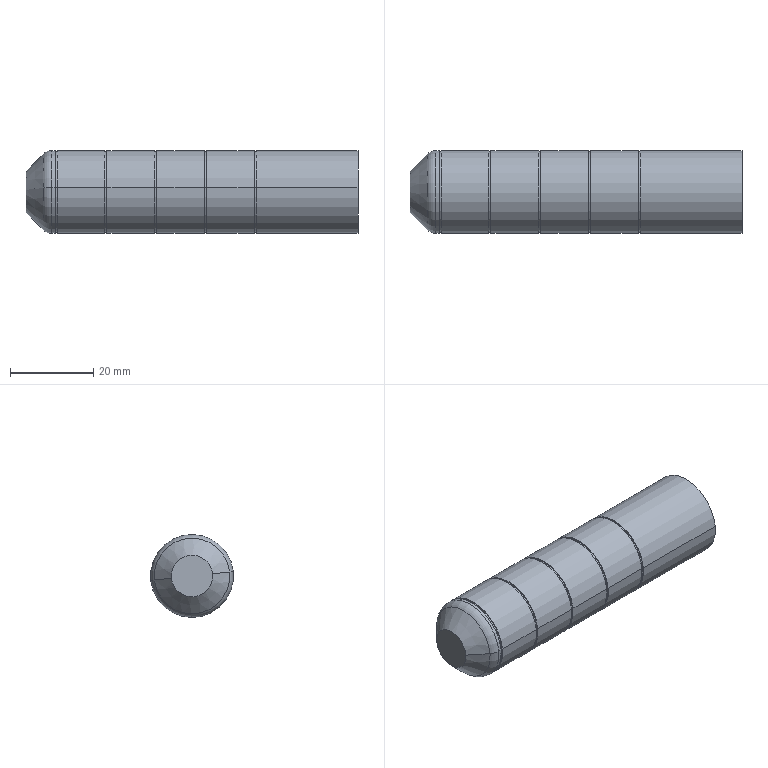Component | SolidWorks | ZN-A-018-2 | 1 solid | 42 faces | box 80 x 20 x 20 mm | volume 23686 mm3 | cylinder 24 | plane 12 | cone 4 | torus 2 | commonest cylinder face diameters 20 x12 19.5 x10 6.8 x2
STEP:
#1=COLOUR_RGB('',0.7922,0.8196,0.9333);
#2=FILL_AREA_STYLE_COLOUR('',#1);
#3=FILL_AREA_STYLE('',(#2));
#4=SURFACE_STYLE_FILL_AREA(#3);
#5=SURFACE_SIDE_STYLE('',(#4));
#6=SURFACE_STYLE_USAGE(.BOTH.,#5);
#7=PRESENTATION_STYLE_ASSIGNMENT((#6));
#8=CARTESIAN_POINT('',(14.356,6.199,4.014));
#9=VERTEX_POINT('',#8);
#10=CARTESIAN_POINT('',(14.356,5.416,4.097));
#11=VERTEX_POINT('',#10);
#12=CARTESIAN_POINT('',(14.356,5.807,4.055));
#13=DIRECTION('',(1.,-0.,0.));
#14=DIRECTION('',(0.,-0.9945,0.1051));
#15=AXIS2_PLACEMENT_3D('',#12,#13,#14);
#16=CIRCLE('',#15,0.3937);
#17=EDGE_CURVE('',#9,#11,#16,.T.);
#18=ORIENTED_EDGE('',*,*,#17,.T.);
#19=CARTESIAN_POINT('',(14.386,5.416,4.097));
#20=VERTEX_POINT('',#19);
#21=CARTESIAN_POINT('',(14.11,5.416,4.097));
#22=DIRECTION('',(1.,-0.,0.));
#23=VECTOR('',#22,39.37);
#24=LINE('',#21,#23);
#25=EDGE_CURVE('',#11,#20,#24,.T.);
#26=ORIENTED_EDGE('',*,*,#25,.T.);
#27=CARTESIAN_POINT('',(14.386,6.199,4.014));
#28=VERTEX_POINT('',#27);
#29=CARTESIAN_POINT('',(14.386,5.807,4.055));
#30=DIRECTION('',(1.,-0.,0.));
#31=DIRECTION('',(0.,0.9945,-0.1051));
#32=AXIS2_PLACEMENT_3D('',#29,#30,#31);
#33=CIRCLE('',#32,0.3937);
#34=EDGE_CURVE('',#28,#20,#33,.T.);
#35=ORIENTED_EDGE('',*,*,#34,.F.);
#36=CARTESIAN_POINT('',(14.11,6.199,4.014));
#37=DIRECTION('',(1.,-0.,0.));
#38=VECTOR('',#37,39.37);
#39=LINE('',#36,#38);
#40=EDGE_CURVE('',#9,#28,#39,.T.);
#41=ORIENTED_EDGE('',*,*,#40,.F.);
#42=EDGE_LOOP('',(#18,#26,#35,#41));
#43=FACE_OUTER_BOUND('',#42,.T.);
#44=CARTESIAN_POINT('',(14.11,5.807,4.055));
#45=DIRECTION('',(1.,-0.,0.));
#46=DIRECTION('',(0.,0.9945,-0.1051));
#47=AXIS2_PLACEMENT_3D('',#44,#45,#46);
#48=CYLINDRICAL_SURFACE('',#47,0.3937);
#49=ADVANCED_FACE('',(#43),#48,.T.);
#50=ORIENTED_EDGE('',*,*,#17,.F.);
#51=CARTESIAN_POINT('',(14.272,6.164,4.017));
#52=VERTEX_POINT('',#51);
#53=CARTESIAN_POINT('',(14.356,6.081,4.026));
#54=DIRECTION('',(-0.,0.1051,0.9945));
#55=DIRECTION('',(0.,-0.9945,0.1051));
#56=AXIS2_PLACEMENT_3D('',#53,#54,#55);
#57=CIRCLE('',#56,0.1181);
#58=EDGE_CURVE('',#9,#52,#57,.T.);
#59=ORIENTED_EDGE('',*,*,#58,.T.);
#60=CARTESIAN_POINT('',(14.272,5.45,4.093));
#61=VERTEX_POINT('',#60);
#62=CARTESIAN_POINT('',(14.272,5.807,4.055));
#63=DIRECTION('',(-1.,0.,-0.));
#64=DIRECTION('',(0.,0.9945,-0.1051));
#65=AXIS2_PLACEMENT_3D('',#62,#63,#64);
#66=CIRCLE('',#65,0.3591);
#67=EDGE_CURVE('',#61,#52,#66,.T.);
#68=ORIENTED_EDGE('',*,*,#67,.F.);
#69=CARTESIAN_POINT('',(14.356,5.533,4.084));
#70=DIRECTION('',(0.,-0.1051,-0.9945));
#71=DIRECTION('',(0.,0.9945,-0.1051));
#72=AXIS2_PLACEMENT_3D('',#69,#70,#71);
#73=CIRCLE('',#72,0.1181);
#74=EDGE_CURVE('',#11,#61,#73,.T.);
#75=ORIENTED_EDGE('',*,*,#74,.F.);
#76=EDGE_LOOP('',(#50,#59,#68,#75));
#77=FACE_OUTER_BOUND('',#76,.T.);
#78=CARTESIAN_POINT('',(14.356,5.807,4.055));
#79=DIRECTION('',(-1.,0.,-0.));
#80=DIRECTION('',(-0.,-0.9945,0.1051));
#81=AXIS2_PLACEMENT_3D('',#78,#79,#80);
#82=TOROIDAL_SURFACE('',#81,0.2756,0.1181);
#83=ADVANCED_FACE('',(#77),#82,.T.);
#84=CARTESIAN_POINT('',(14.11,5.611,4.076));
#85=VERTEX_POINT('',#84);
#86=CARTESIAN_POINT('',(14.11,6.003,4.034));
#87=VERTEX_POINT('',#86);
#88=CARTESIAN_POINT('',(14.11,5.807,4.055));
#89=DIRECTION('',(-1.,0.,-0.));
#90=DIRECTION('',(0.,-0.9945,0.1051));
#91=AXIS2_PLACEMENT_3D('',#88,#89,#90);
#92=CIRCLE('',#91,0.1969);
#93=EDGE_CURVE('',#85,#87,#92,.T.);
#94=ORIENTED_EDGE('',*,*,#93,.F.);
#95=CARTESIAN_POINT('',(14.11,5.611,4.076));
#96=DIRECTION('',(0.7071,-0.7032,0.07433));
#97=VECTOR('',#96,39.37);
#98=LINE('',#95,#97);
#99=EDGE_CURVE('',#85,#61,#98,.T.);
#100=ORIENTED_EDGE('',*,*,#99,.T.);
#101=ORIENTED_EDGE('',*,*,#67,.T.);
#102=CARTESIAN_POINT('',(14.11,6.003,4.034));
#103=DIRECTION('',(0.7071,0.7032,-0.07433));
#104=VECTOR('',#103,39.37);
#105=LINE('',#102,#104);
#106=EDGE_CURVE('',#87,#52,#105,.T.);
#107=ORIENTED_EDGE('',*,*,#106,.F.);
#108=EDGE_LOOP('',(#94,#100,#101,#107));
#109=FACE_OUTER_BOUND('',#108,.T.);
#110=CARTESIAN_POINT('',(14.11,5.807,4.055));
#111=DIRECTION('',(1.,-0.,0.));
#112=DIRECTION('',(0.,0.9945,-0.1051));
#113=AXIS2_PLACEMENT_3D('',#110,#111,#112);
#114=CONICAL_SURFACE('',#113,0.1969,0.7854);
#115=ADVANCED_FACE('',(#109),#114,.T.);
#116=CARTESIAN_POINT('',(14.405,6.189,4.015));
#117=VERTEX_POINT('',#116);
#118=CARTESIAN_POINT('',(14.405,5.425,4.095));
#119=VERTEX_POINT('',#118);
#120=CARTESIAN_POINT('',(14.405,5.807,4.055));
#121=DIRECTION('',(1.,-0.,0.));
#122=DIRECTION('',(0.,0.9945,-0.1051));
#123=AXIS2_PLACEMENT_3D('',#120,#121,#122);
#124=CIRCLE('',#123,0.3839);
#125=EDGE_CURVE('',#117,#119,#124,.T.);
#126=ORIENTED_EDGE('',*,*,#125,.F.);
#127=CARTESIAN_POINT('',(14.386,6.189,4.015));
#128=VERTEX_POINT('',#127);
#129=CARTESIAN_POINT('',(14.405,6.189,4.015));
#130=DIRECTION('',(-1.,0.,-0.));
#131=VECTOR('',#130,39.37);
#132=LINE('',#129,#131);
#133=EDGE_CURVE('',#117,#128,#132,.T.);
#134=ORIENTED_EDGE('',*,*,#133,.T.);
#135=CARTESIAN_POINT('',(14.386,5.425,4.095));
#136=VERTEX_POINT('',#135);
#137=CARTESIAN_POINT('',(14.386,5.807,4.055));
#138=DIRECTION('',(1.,-0.,0.));
#139=DIRECTION('',(0.,0.9945,-0.1051));
#140=AXIS2_PLACEMENT_3D('',#137,#138,#139);
#141=CIRCLE('',#140,0.3839);
#142=EDGE_CURVE('',#128,#136,#141,.T.);
#143=ORIENTED_EDGE('',*,*,#142,.T.);
#144=CARTESIAN_POINT('',(14.405,5.425,4.095));
#145=DIRECTION('',(-1.,0.,-0.));
#146=VECTOR('',#145,39.37);
#147=LINE('',#144,#146);
#148=EDGE_CURVE('',#119,#136,#147,.T.);
#149=ORIENTED_EDGE('',*,*,#148,.F.);
#150=EDGE_LOOP('',(#126,#134,#143,#149));
#151=FACE_OUTER_BOUND('',#150,.T.);
#152=CARTESIAN_POINT('',(14.405,5.807,4.055));
#153=DIRECTION('',(-1.,0.,-0.));
#154=DIRECTION('',(0.,-0.9945,0.1051));
#155=AXIS2_PLACEMENT_3D('',#152,#153,#154);
#156=CYLINDRICAL_SURFACE('',#155,0.3839);
#157=ADVANCED_FACE('',(#151),#156,.T.);
#158=CARTESIAN_POINT('',(14.405,6.199,4.014));
#159=VERTEX_POINT('',#158);
#160=CARTESIAN_POINT('',(14.405,5.416,4.097));
#161=VERTEX_POINT('',#160);
#162=CARTESIAN_POINT('',(14.405,5.807,4.055));
#163=DIRECTION('',(1.,-0.,0.));
#164=DIRECTION('',(0.,0.9945,-0.1051));
#165=AXIS2_PLACEMENT_3D('',#162,#163,#164);
#166=CIRCLE('',#165,0.3937);
#167=EDGE_CURVE('',#159,#161,#166,.T.);
#168=ORIENTED_EDGE('',*,*,#167,.T.);
#169=CARTESIAN_POINT('',(14.858,5.416,4.097));
#170=VERTEX_POINT('',#169);
#171=CARTESIAN_POINT('',(14.11,5.416,4.097));
#172=DIRECTION('',(1.,-0.,0.));
#173=VECTOR('',#172,39.37);
#174=LINE('',#171,#173);
#175=EDGE_CURVE('',#161,#170,#174,.T.);
#176=ORIENTED_EDGE('',*,*,#175,.T.);
#177=CARTESIAN_POINT('',(14.858,6.199,4.014));
#178=VERTEX_POINT('',#177);
#179=CARTESIAN_POINT('',(14.858,5.807,4.055));
#180=DIRECTION('',(1.,-0.,0.));
#181=DIRECTION('',(0.,0.9945,-0.1051));
#182=AXIS2_PLACEMENT_3D('',#179,#180,#181);
#183=CIRCLE('',#182,0.3937);
#184=EDGE_CURVE('',#178,#170,#183,.T.);
#185=ORIENTED_EDGE('',*,*,#184,.F.);
#186=CARTESIAN_POINT('',(14.11,6.199,4.014));
#187=DIRECTION('',(1.,-0.,0.));
#188=VECTOR('',#187,39.37);
#189=LINE('',#186,#188);
#190=EDGE_CURVE('',#159,#178,#189,.T.);
#191=ORIENTED_EDGE('',*,*,#190,.F.);
#192=EDGE_LOOP('',(#168,#176,#185,#191));
#193=FACE_OUTER_BOUND('',#192,.T.);
#194=CARTESIAN_POINT('',(14.11,5.807,4.055));
#195=DIRECTION('',(1.,-0.,0.));
#196=DIRECTION('',(0.,0.9945,-0.1051));
#197=AXIS2_PLACEMENT_3D('',#194,#195,#196);
#198=CYLINDRICAL_SURFACE('',#197,0.3937);
#199=ADVANCED_FACE('',(#193),#198,.T.);
#200=CARTESIAN_POINT('',(14.878,6.189,4.015));
#201=VERTEX_POINT('',#200);
#202=CARTESIAN_POINT('',(14.878,5.425,4.095));
#203=VERTEX_POINT('',#202);
#204=CARTESIAN_POINT('',(14.878,5.807,4.055));
#205=DIRECTION('',(1.,-0.,0.));
#206=DIRECTION('',(0.,0.9945,-0.1051));
#207=AXIS2_PLACEMENT_3D('',#204,#205,#206);
#208=CIRCLE('',#207,0.3839);
#209=EDGE_CURVE('',#201,#203,#208,.T.);
#210=ORIENTED_EDGE('',*,*,#209,.F.);
#211=CARTESIAN_POINT('',(14.858,6.189,4.015));
#212=VERTEX_POINT('',#211);
#213=CARTESIAN_POINT('',(14.878,6.189,4.015));
#214=DIRECTION('',(-1.,0.,-0.));
#215=VECTOR('',#214,39.37);
#216=LINE('',#213,#215);
#217=EDGE_CURVE('',#201,#212,#216,.T.);
#218=ORIENTED_EDGE('',*,*,#217,.T.);
#219=CARTESIAN_POINT('',(14.858,5.425,4.095));
#220=VERTEX_POINT('',#219);
#221=CARTESIAN_POINT('',(14.858,5.807,4.055));
#222=DIRECTION('',(1.,-0.,0.));
#223=DIRECTION('',(0.,0.9945,-0.1051));
#224=AXIS2_PLACEMENT_3D('',#221,#222,#223);
#225=CIRCLE('',#224,0.3839);
#226=EDGE_CURVE('',#212,#220,#225,.T.);
#227=ORIENTED_EDGE('',*,*,#226,.T.);
#228=CARTESIAN_POINT('',(14.878,5.425,4.095));
#229=DIRECTION('',(-1.,0.,-0.));
#230=VECTOR('',#229,39.37);
#231=LINE('',#228,#230);
#232=EDGE_CURVE('',#203,#220,#231,.T.);
#233=ORIENTED_EDGE('',*,*,#232,.F.);
#234=EDGE_LOOP('',(#210,#218,#227,#233));
#235=FACE_OUTER_BOUND('',#234,.T.);
#236=CARTESIAN_POINT('',(14.878,5.807,4.055));
#237=DIRECTION('',(-1.,0.,-0.));
#238=DIRECTION('',(0.,-0.9945,0.1051));
#239=AXIS2_PLACEMENT_3D('',#236,#237,#238);
#240=CYLINDRICAL_SURFACE('',#239,0.3839);
#241=ADVANCED_FACE('',(#235),#240,.T.);
#242=CARTESIAN_POINT('',(14.878,6.199,4.014));
#243=VERTEX_POINT('',#242);
#244=CARTESIAN_POINT('',(14.878,5.416,4.097));
#245=VERTEX_POINT('',#244);
#246=CARTESIAN_POINT('',(14.878,5.807,4.055));
#247=DIRECTION('',(1.,-0.,0.));
#248=DIRECTION('',(0.,0.9945,-0.1051));
#249=AXIS2_PLACEMENT_3D('',#246,#247,#248);
#250=CIRCLE('',#249,0.3937);
#251=EDGE_CURVE('',#243,#245,#250,.T.);
#252=ORIENTED_EDGE('',*,*,#251,.T.);
#253=CARTESIAN_POINT('',(15.33,5.416,4.097));
#254=VERTEX_POINT('',#253);
#255=CARTESIAN_POINT('',(14.11,5.416,4.097));
#256=DIRECTION('',(1.,-0.,0.));
#257=VECTOR('',#256,39.37);
#258=LINE('',#255,#257);
#259=EDGE_CURVE('',#245,#254,#258,.T.);
#260=ORIENTED_EDGE('',*,*,#259,.T.);
#261=CARTESIAN_POINT('',(15.33,6.199,4.014));
#262=VERTEX_POINT('',#261);
#263=CARTESIAN_POINT('',(15.33,5.807,4.055));
#264=DIRECTION('',(1.,-0.,0.));
#265=DIRECTION('',(0.,0.9945,-0.1051));
#266=AXIS2_PLACEMENT_3D('',#263,#264,#265);
#267=CIRCLE('',#266,0.3937);
#268=EDGE_CURVE('',#262,#254,#267,.T.);
#269=ORIENTED_EDGE('',*,*,#268,.F.);
#270=CARTESIAN_POINT('',(14.11,6.199,4.014));
#271=DIRECTION('',(1.,-0.,0.));
#272=VECTOR('',#271,39.37);
#273=LINE('',#270,#272);
#274=EDGE_CURVE('',#243,#262,#273,.T.);
#275=ORIENTED_EDGE('',*,*,#274,.F.);
#276=EDGE_LOOP('',(#252,#260,#269,#275));
#277=FACE_OUTER_BOUND('',#276,.T.);
#278=CARTESIAN_POINT('',(14.11,5.807,4.055));
#279=DIRECTION('',(1.,-0.,0.));
#280=DIRECTION('',(0.,0.9945,-0.1051));
#281=AXIS2_PLACEMENT_3D('',#278,#279,#280);
#282=CYLINDRICAL_SURFACE('',#281,0.3937);
#283=ADVANCED_FACE('',(#277),#282,.T.);
#284=CARTESIAN_POINT('',(15.35,6.189,4.015));
#285=VERTEX_POINT('',#284);
#286=CARTESIAN_POINT('',(15.35,5.425,4.095));
#287=VERTEX_POINT('',#286);
#288=CARTESIAN_POINT('',(15.35,5.807,4.055));
#289=DIRECTION('',(1.,-0.,0.));
#290=DIRECTION('',(0.,0.9945,-0.1051));
#291=AXIS2_PLACEMENT_3D('',#288,#289,#290);
#292=CIRCLE('',#291,0.3839);
#293=EDGE_CURVE('',#285,#287,#292,.T.);
#294=ORIENTED_EDGE('',*,*,#293,.F.);
#295=CARTESIAN_POINT('',(15.33,6.189,4.015));
#296=VERTEX_POINT('',#295);
#297=CARTESIAN_POINT('',(15.35,6.189,4.015));
#298=DIRECTION('',(-1.,0.,-0.));
#299=VECTOR('',#298,39.37);
#300=LINE('',#297,#299);
#301=EDGE_CURVE('',#285,#296,#300,.T.);
#302=ORIENTED_EDGE('',*,*,#301,.T.);
#303=CARTESIAN_POINT('',(15.33,5.425,4.095));
#304=VERTEX_POINT('',#303);
#305=CARTESIAN_POINT('',(15.33,5.807,4.055));
#306=DIRECTION('',(1.,-0.,0.));
#307=DIRECTION('',(0.,0.9945,-0.1051));
#308=AXIS2_PLACEMENT_3D('',#305,#306,#307);
#309=CIRCLE('',#308,0.3839);
#310=EDGE_CURVE('',#296,#304,#309,.T.);
#311=ORIENTED_EDGE('',*,*,#310,.T.);
#312=CARTESIAN_POINT('',(15.35,5.425,4.095));
#313=DIRECTION('',(-1.,0.,-0.));
#314=VECTOR('',#313,39.37);
#315=LINE('',#312,#314);
#316=EDGE_CURVE('',#287,#304,#315,.T.);
#317=ORIENTED_EDGE('',*,*,#316,.F.);
#318=EDGE_LOOP('',(#294,#302,#311,#317));
#319=FACE_OUTER_BOUND('',#318,.T.);
#320=CARTESIAN_POINT('',(15.35,5.807,4.055));
#321=DIRECTION('',(-1.,0.,-0.));
#322=DIRECTION('',(0.,-0.9945,0.1051));
#323=AXIS2_PLACEMENT_3D('',#320,#321,#322);
#324=CYLINDRICAL_SURFACE('',#323,0.3839);
#325=ADVANCED_FACE('',(#319),#324,.T.);
#326=CARTESIAN_POINT('',(15.35,6.199,4.014));
#327=VERTEX_POINT('',#326);
#328=CARTESIAN_POINT('',(15.35,5.416,4.097));
#329=VERTEX_POINT('',#328);
#330=CARTESIAN_POINT('',(15.35,5.807,4.055));
#331=DIRECTION('',(1.,-0.,0.));
#332=DIRECTION('',(0.,0.9945,-0.1051));
#333=AXIS2_PLACEMENT_3D('',#330,#331,#332);
#334=CIRCLE('',#333,0.3937);
#335=EDGE_CURVE('',#327,#329,#334,.T.);
#336=ORIENTED_EDGE('',*,*,#335,.T.);
#337=CARTESIAN_POINT('',(15.803,5.416,4.097));
#338=VERTEX_POINT('',#337);
#339=CARTESIAN_POINT('',(14.11,5.416,4.097));
#340=DIRECTION('',(1.,-0.,0.));
#341=VECTOR('',#340,39.37);
#342=LINE('',#339,#341);
#343=EDGE_CURVE('',#329,#338,#342,.T.);
#344=ORIENTED_EDGE('',*,*,#343,.T.);
#345=CARTESIAN_POINT('',(15.803,6.199,4.014));
#346=VERTEX_POINT('',#345);
#347=CARTESIAN_POINT('',(15.803,5.807,4.055));
#348=DIRECTION('',(1.,-0.,0.));
#349=DIRECTION('',(0.,0.9945,-0.1051));
#350=AXIS2_PLACEMENT_3D('',#347,#348,#349);
#351=CIRCLE('',#350,0.3937);
#352=EDGE_CURVE('',#346,#338,#351,.T.);
#353=ORIENTED_EDGE('',*,*,#352,.F.);
#354=CARTESIAN_POINT('',(14.11,6.199,4.014));
#355=DIRECTION('',(1.,-0.,0.));
#356=VECTOR('',#355,39.37);
#357=LINE('',#354,#356);
#358=EDGE_CURVE('',#327,#346,#357,.T.);
#359=ORIENTED_EDGE('',*,*,#358,.F.);
#360=EDGE_LOOP('',(#336,#344,#353,#359));
#361=FACE_OUTER_BOUND('',#360,.T.);
#362=CARTESIAN_POINT('',(14.11,5.807,4.055));
#363=DIRECTION('',(1.,-0.,0.));
#364=DIRECTION('',(0.,0.9945,-0.1051));
#365=AXIS2_PLACEMENT_3D('',#362,#363,#364);
#366=CYLINDRICAL_SURFACE('',#365,0.3937);
#367=ADVANCED_FACE('',(#361),#366,.T.);
#368=CARTESIAN_POINT('',(15.823,6.189,4.015));
#369=VERTEX_POINT('',#368);
#370=CARTESIAN_POINT('',(15.823,5.425,4.095));
#371=VERTEX_POINT('',#370);
#372=CARTESIAN_POINT('',(15.823,5.807,4.055));
#373=DIRECTION('',(1.,-0.,0.));
#374=DIRECTION('',(0.,0.9945,-0.1051));
#375=AXIS2_PLACEMENT_3D('',#372,#373,#374);
#376=CIRCLE('',#375,0.3839);
#377=EDGE_CURVE('',#369,#371,#376,.T.);
#378=ORIENTED_EDGE('',*,*,#377,.F.);
#379=CARTESIAN_POINT('',(15.803,6.189,4.015));
#380=VERTEX_POINT('',#379);
#381=CARTESIAN_POINT('',(15.823,6.189,4.015));
#382=DIRECTION('',(-1.,0.,-0.));
#383=VECTOR('',#382,39.37);
#384=LINE('',#381,#383);
#385=EDGE_CURVE('',#369,#380,#384,.T.);
#386=ORIENTED_EDGE('',*,*,#385,.T.);
#387=CARTESIAN_POINT('',(15.803,5.425,4.095));
#388=VERTEX_POINT('',#387);
#389=CARTESIAN_POINT('',(15.803,5.807,4.055));
#390=DIRECTION('',(1.,-0.,0.));
#391=DIRECTION('',(0.,0.9945,-0.1051));
#392=AXIS2_PLACEMENT_3D('',#389,#390,#391);
#393=CIRCLE('',#392,0.3839);
#394=EDGE_CURVE('',#380,#388,#393,.T.);
#395=ORIENTED_EDGE('',*,*,#394,.T.);
#396=CARTESIAN_POINT('',(15.823,5.425,4.095));
#397=DIRECTION('',(-1.,0.,-0.));
#398=VECTOR('',#397,39.37);
#399=LINE('',#396,#398);
#400=EDGE_CURVE('',#371,#388,#399,.T.);
#401=ORIENTED_EDGE('',*,*,#400,.F.);
#402=EDGE_LOOP('',(#378,#386,#395,#401));
#403=FACE_OUTER_BOUND('',#402,.T.);
#404=CARTESIAN_POINT('',(15.823,5.807,4.055));
#405=DIRECTION('',(-1.,0.,-0.));
#406=DIRECTION('',(0.,-0.9945,0.1051));
#407=AXIS2_PLACEMENT_3D('',#404,#405,#406);
#408=CYLINDRICAL_SURFACE('',#407,0.3839);
#409=ADVANCED_FACE('',(#403),#408,.T.);
#410=CARTESIAN_POINT('',(15.823,6.199,4.014));
#411=VERTEX_POINT('',#410);
#412=CARTESIAN_POINT('',(15.823,5.416,4.097));
#413=VERTEX_POINT('',#412);
#414=CARTESIAN_POINT('',(15.823,5.807,4.055));
#415=DIRECTION('',(1.,-0.,0.));
#416=DIRECTION('',(0.,0.9945,-0.1051));
#417=AXIS2_PLACEMENT_3D('',#414,#415,#416);
#418=CIRCLE('',#417,0.3937);
#419=EDGE_CURVE('',#411,#413,#418,.T.);
#420=ORIENTED_EDGE('',*,*,#419,.T.);
#421=CARTESIAN_POINT('',(16.275,5.416,4.097));
#422=VERTEX_POINT('',#421);
#423=CARTESIAN_POINT('',(14.11,5.416,4.097));
#424=DIRECTION('',(1.,-0.,0.));
#425=VECTOR('',#424,39.37);
#426=LINE('',#423,#425);
#427=EDGE_CURVE('',#413,#422,#426,.T.);
#428=ORIENTED_EDGE('',*,*,#427,.T.);
#429=CARTESIAN_POINT('',(16.275,6.199,4.014));
#430=VERTEX_POINT('',#429);
#431=CARTESIAN_POINT('',(16.275,5.807,4.055));
#432=DIRECTION('',(1.,-0.,0.));
#433=DIRECTION('',(0.,0.9945,-0.1051));
#434=AXIS2_PLACEMENT_3D('',#431,#432,#433);
#435=CIRCLE('',#434,0.3937);
#436=EDGE_CURVE('',#430,#422,#435,.T.);
#437=ORIENTED_EDGE('',*,*,#436,.F.);
#438=CARTESIAN_POINT('',(14.11,6.199,4.014));
#439=DIRECTION('',(1.,-0.,0.));
#440=VECTOR('',#439,39.37);
#441=LINE('',#438,#440);
#442=EDGE_CURVE('',#411,#430,#441,.T.);
#443=ORIENTED_EDGE('',*,*,#442,.F.);
#444=EDGE_LOOP('',(#420,#428,#437,#443));
#445=FACE_OUTER_BOUND('',#444,.T.);
#446=CARTESIAN_POINT('',(14.11,5.807,4.055));
#447=DIRECTION('',(1.,-0.,0.));
#448=DIRECTION('',(0.,0.9945,-0.1051));
#449=AXIS2_PLACEMENT_3D('',#446,#447,#448);
#450=CYLINDRICAL_SURFACE('',#449,0.3937);
#451=ADVANCED_FACE('',(#445),#450,.T.);
#452=CARTESIAN_POINT('',(16.295,6.189,4.015));
#453=VERTEX_POINT('',#452);
#454=CARTESIAN_POINT('',(16.295,5.425,4.095));
#455=VERTEX_POINT('',#454);
#456=CARTESIAN_POINT('',(16.295,5.807,4.055));
#457=DIRECTION('',(1.,-0.,0.));
#458=DIRECTION('',(0.,0.9945,-0.1051));
#459=AXIS2_PLACEMENT_3D('',#456,#457,#458);
#460=CIRCLE('',#459,0.3839);
#461=EDGE_CURVE('',#453,#455,#460,.T.);
#462=ORIENTED_EDGE('',*,*,#461,.F.);
#463=CARTESIAN_POINT('',(16.275,6.189,4.015));
#464=VERTEX_POINT('',#463);
#465=CARTESIAN_POINT('',(16.295,6.189,4.015));
#466=DIRECTION('',(-1.,0.,-0.));
#467=VECTOR('',#466,39.37);
#468=LINE('',#465,#467);
#469=EDGE_CURVE('',#453,#464,#468,.T.);
#470=ORIENTED_EDGE('',*,*,#469,.T.);
#471=CARTESIAN_POINT('',(16.275,5.425,4.095));
#472=VERTEX_POINT('',#471);
#473=CARTESIAN_POINT('',(16.275,5.807,4.055));
#474=DIRECTION('',(1.,-0.,0.));
#475=DIRECTION('',(0.,0.9945,-0.1051));
#476=AXIS2_PLACEMENT_3D('',#473,#474,#475);
#477=CIRCLE('',#476,0.3839);
#478=EDGE_CURVE('',#464,#472,#477,.T.);
#479=ORIENTED_EDGE('',*,*,#478,.T.);
#480=CARTESIAN_POINT('',(16.295,5.425,4.095));
#481=DIRECTION('',(-1.,0.,-0.));
#482=VECTOR('',#481,39.37);
#483=LINE('',#480,#482);
#484=EDGE_CURVE('',#455,#472,#483,.T.);
#485=ORIENTED_EDGE('',*,*,#484,.F.);
#486=EDGE_LOOP('',(#462,#470,#479,#485));
#487=FACE_OUTER_BOUND('',#486,.T.);
#488=CARTESIAN_POINT('',(16.295,5.807,4.055));
#489=DIRECTION('',(-1.,0.,-0.));
#490=DIRECTION('',(0.,-0.9945,0.1051));
#491=AXIS2_PLACEMENT_3D('',#488,#489,#490);
#492=CYLINDRICAL_SURFACE('',#491,0.3839);
#493=ADVANCED_FACE('',(#487),#492,.T.);
#494=CARTESIAN_POINT('',(16.482,5.674,4.069));
#495=VERTEX_POINT('',#494);
#496=CARTESIAN_POINT('',(16.482,5.94,4.041));
#497=VERTEX_POINT('',#496);
#498=CARTESIAN_POINT('',(16.482,5.807,4.055));
#499=DIRECTION('',(1.,-0.,0.));
#500=DIRECTION('',(0.,0.9945,-0.1051));
#501=AXIS2_PLACEMENT_3D('',#498,#499,#500);
#502=CIRCLE('',#501,0.1339);
#503=EDGE_CURVE('',#495,#497,#502,.T.);
#504=ORIENTED_EDGE('',*,*,#503,.F.);
#505=CARTESIAN_POINT('',(17.26,5.674,4.069));
#506=VERTEX_POINT('',#505);
#507=CARTESIAN_POINT('',(17.26,5.674,4.069));
#508=DIRECTION('',(1.,-0.,0.));
#509=VECTOR('',#508,39.37);
#510=LINE('',#507,#509);
#511=EDGE_CURVE('',#495,#506,#510,.T.);
#512=ORIENTED_EDGE('',*,*,#511,.T.);
#513=CARTESIAN_POINT('',(17.26,5.94,4.041));
#514=VERTEX_POINT('',#513);
#515=CARTESIAN_POINT('',(17.26,5.807,4.055));
#516=DIRECTION('',(1.,-0.,0.));
#517=DIRECTION('',(0.,0.9945,-0.1051));
#518=AXIS2_PLACEMENT_3D('',#515,#516,#517);
#519=CIRCLE('',#518,0.1339);
#520=EDGE_CURVE('',#506,#514,#519,.T.);
#521=ORIENTED_EDGE('',*,*,#520,.T.);
#522=CARTESIAN_POINT('',(17.26,5.94,4.041));
#523=DIRECTION('',(1.,-0.,0.));
#524=VECTOR('',#523,39.37);
#525=LINE('',#522,#524);
#526=EDGE_CURVE('',#497,#514,#525,.T.);
#527=ORIENTED_EDGE('',*,*,#526,.F.);
#528=EDGE_LOOP('',(#504,#512,#521,#527));
#529=FACE_OUTER_BOUND('',#528,.T.);
#530=CARTESIAN_POINT('',(17.26,5.807,4.055));
#531=DIRECTION('',(1.,-0.,0.));
#532=DIRECTION('',(0.,0.9945,-0.1051));
#533=AXIS2_PLACEMENT_3D('',#530,#531,#532);
#534=CYLINDRICAL_SURFACE('',#533,0.1339);
#535=ADVANCED_FACE('',(#529),#534,.F.);
#536=CARTESIAN_POINT('',(16.402,5.807,4.055));
#537=VERTEX_POINT('',#536);
#538=CARTESIAN_POINT('',(16.482,5.94,4.041));
#539=DIRECTION('',(0.515,0.8524,-0.0901));
#540=VECTOR('',#539,39.37);
#541=LINE('',#538,#540);
#542=EDGE_CURVE('',#537,#497,#541,.T.);
#543=ORIENTED_EDGE('',*,*,#542,.F.);
#544=CARTESIAN_POINT('',(16.482,5.674,4.069));
#545=DIRECTION('',(0.515,-0.8524,0.0901));
#546=VECTOR('',#545,39.37);
#547=LINE('',#544,#546);
#548=EDGE_CURVE('',#537,#495,#547,.T.);
#549=ORIENTED_EDGE('',*,*,#548,.T.);
#550=ORIENTED_EDGE('',*,*,#503,.T.);
#551=EDGE_LOOP('',(#543,#549,#550));
#552=FACE_OUTER_BOUND('',#551,.T.);
#553=CARTESIAN_POINT('',(16.482,5.807,4.055));
#554=DIRECTION('',(1.,-0.,0.));
#555=DIRECTION('',(0.,0.9945,-0.1051));
#556=AXIS2_PLACEMENT_3D('',#553,#554,#555);
#557=CONICAL_SURFACE('',#556,0.1339,1.03);
#558=ADVANCED_FACE('',(#552),#557,.F.);
#559=CARTESIAN_POINT('',(16.295,6.199,4.014));
#560=VERTEX_POINT('',#559);
#561=CARTESIAN_POINT('',(16.295,5.416,4.097));
#562=VERTEX_POINT('',#561);
#563=CARTESIAN_POINT('',(16.295,5.807,4.055));
#564=DIRECTION('',(1.,-0.,0.));
#565=DIRECTION('',(0.,0.9945,-0.1051));
#566=AXIS2_PLACEMENT_3D('',#563,#564,#565);
#567=CIRCLE('',#566,0.3937);
#568=EDGE_CURVE('',#560,#562,#567,.T.);
#569=ORIENTED_EDGE('',*,*,#568,.T.);
#570=CARTESIAN_POINT('',(17.26,5.416,4.097));
#571=VERTEX_POINT('',#570);
#572=CARTESIAN_POINT('',(14.11,5.416,4.097));
#573=DIRECTION('',(1.,-0.,0.));
#574=VECTOR('',#573,39.37);
#575=LINE('',#572,#574);
#576=EDGE_CURVE('',#562,#571,#575,.T.);
#577=ORIENTED_EDGE('',*,*,#576,.T.);
#578=CARTESIAN_POINT('',(17.26,6.199,4.014));
#579=VERTEX_POINT('',#578);
#580=CARTESIAN_POINT('',(17.26,5.807,4.055));
#581=DIRECTION('',(-1.,0.,-0.));
#582=DIRECTION('',(0.,-0.9945,0.1051));
#583=AXIS2_PLACEMENT_3D('',#580,#581,#582);
#584=CIRCLE('',#583,0.3937);
#585=EDGE_CURVE('',#571,#579,#584,.T.);
#586=ORIENTED_EDGE('',*,*,#585,.T.);
#587=CARTESIAN_POINT('',(14.11,6.199,4.014));
#588=DIRECTION('',(1.,-0.,0.));
#589=VECTOR('',#588,39.37);
#590=LINE('',#587,#589);
#591=EDGE_CURVE('',#560,#579,#590,.T.);
#592=ORIENTED_EDGE('',*,*,#591,.F.);
#593=EDGE_LOOP('',(#569,#577,#586,#592));
#594=FACE_OUTER_BOUND('',#593,.T.);
#595=CARTESIAN_POINT('',(14.11,5.807,4.055));
#596=DIRECTION('',(1.,-0.,0.));
#597=DIRECTION('',(0.,0.9945,-0.1051));
#598=AXIS2_PLACEMENT_3D('',#595,#596,#597);
#599=CYLINDRICAL_SURFACE('',#598,0.3937);
#600=ADVANCED_FACE('',(#594),#599,.T.);
#601=ORIENTED_EDGE('',*,*,#576,.F.);
#602=CARTESIAN_POINT('',(16.295,5.807,4.055));
#603=DIRECTION('',(1.,-0.,0.));
#604=DIRECTION('',(0.,0.9945,-0.1051));
#605=AXIS2_PLACEMENT_3D('',#602,#603,#604);
#606=CIRCLE('',#605,0.3937);
#607=EDGE_CURVE('',#562,#560,#606,.T.);
#608=ORIENTED_EDGE('',*,*,#607,.T.);
#609=ORIENTED_EDGE('',*,*,#591,.T.);
#610=CARTESIAN_POINT('',(17.26,5.807,4.055));
#611=DIRECTION('',(-1.,0.,-0.));
#612=DIRECTION('',(0.,-0.9945,0.1051));
#613=AXIS2_PLACEMENT_3D('',#610,#611,#612);
#614=CIRCLE('',#613,0.3937);
#615=EDGE_CURVE('',#579,#571,#614,.T.);
#616=ORIENTED_EDGE('',*,*,#615,.T.);
#617=EDGE_LOOP('',(#601,#608,#609,#616));
#618=FACE_OUTER_BOUND('',#617,.T.);
#619=CARTESIAN_POINT('',(14.11,5.807,4.055));
#620=DIRECTION('',(1.,-0.,0.));
#621=DIRECTION('',(0.,0.9945,-0.1051));
#622=AXIS2_PLACEMENT_3D('',#619,#620,#621);
#623=CYLINDRICAL_SURFACE('',#622,0.3937);
#624=ADVANCED_FACE('',(#618),#623,.T.);
#625=CARTESIAN_POINT('',(17.26,5.807,4.055));
#626=DIRECTION('',(1.,-0.,0.));
#627=DIRECTION('',(0.,0.9945,-0.1051));
#628=AXIS2_PLACEMENT_3D('',#625,#626,#627);
#629=CIRCLE('',#628,0.1339);
#630=EDGE_CURVE('',#514,#506,#629,.T.);
#631=ORIENTED_EDGE('',*,*,#630,.F.);
#632=ORIENTED_EDGE('',*,*,#520,.F.);
#633=EDGE_LOOP('',(#631,#632));
#634=FACE_BOUND('',#633,.T.);
#635=ORIENTED_EDGE('',*,*,#615,.F.);
#636=ORIENTED_EDGE('',*,*,#585,.F.);
#637=EDGE_LOOP('',(#635,#636));
#638=FACE_OUTER_BOUND('',#637,.T.);
#639=CARTESIAN_POINT('',(17.26,5.807,4.055));
#640=DIRECTION('',(-1.,0.,-0.));
#641=DIRECTION('',(-0.,-0.9945,0.1051));
#642=AXIS2_PLACEMENT_3D('',#639,#640,#641);
#643=PLANE('',#642);
#644=ADVANCED_FACE('',(#634,#638),#643,.F.);
#645=ORIENTED_EDGE('',*,*,#548,.F.);
#646=ORIENTED_EDGE('',*,*,#542,.T.);
#647=CARTESIAN_POINT('',(16.482,5.807,4.055));
#648=DIRECTION('',(1.,-0.,0.));
#649=DIRECTION('',(0.,0.9945,-0.1051));
#650=AXIS2_PLACEMENT_3D('',#647,#648,#649);
#651=CIRCLE('',#650,0.1339);
#652=EDGE_CURVE('',#497,#495,#651,.T.);
#653=ORIENTED_EDGE('',*,*,#652,.T.);
#654=EDGE_LOOP('',(#645,#646,#653));
#655=FACE_OUTER_BOUND('',#654,.T.);
#656=CARTESIAN_POINT('',(16.482,5.807,4.055));
#657=DIRECTION('',(1.,-0.,0.));
#658=DIRECTION('',(0.,0.9945,-0.1051));
#659=AXIS2_PLACEMENT_3D('',#656,#657,#658);
#660=CONICAL_SURFACE('',#659,0.1339,1.03);
#661=ADVANCED_FACE('',(#655),#660,.F.);
#662=ORIENTED_EDGE('',*,*,#511,.F.);
#663=ORIENTED_EDGE('',*,*,#652,.F.);
#664=ORIENTED_EDGE('',*,*,#526,.T.);
#665=ORIENTED_EDGE('',*,*,#630,.T.);
#666=EDGE_LOOP('',(#662,#663,#664,#665));
#667=FACE_OUTER_BOUND('',#666,.T.);
#668=CARTESIAN_POINT('',(17.26,5.807,4.055));
#669=DIRECTION('',(1.,-0.,0.));
#670=DIRECTION('',(0.,0.9945,-0.1051));
#671=AXIS2_PLACEMENT_3D('',#668,#669,#670);
#672=CYLINDRICAL_SURFACE('',#671,0.1339);
#673=ADVANCED_FACE('',(#667),#672,.F.);
#674=ORIENTED_EDGE('',*,*,#568,.F.);
#675=ORIENTED_EDGE('',*,*,#607,.F.);
#676=EDGE_LOOP('',(#674,#675));
#677=FACE_OUTER_BOUND('',#676,.T.);
#678=CARTESIAN_POINT('',(16.295,5.807,4.055));
#679=DIRECTION('',(1.,-0.,0.));
#680=DIRECTION('',(0.,0.9945,-0.1051));
#681=AXIS2_PLACEMENT_3D('',#678,#679,#680);
#682=CIRCLE('',#681,0.3839);
#683=EDGE_CURVE('',#455,#453,#682,.T.);
#684=ORIENTED_EDGE('',*,*,#683,.T.);
#685=ORIENTED_EDGE('',*,*,#461,.T.);
#686=EDGE_LOOP('',(#684,#685));
#687=FACE_BOUND('',#686,.T.);
#688=CARTESIAN_POINT('',(16.295,5.807,4.055));
#689=DIRECTION('',(1.,-0.,0.));
#690=DIRECTION('',(0.,0.9945,-0.1051));
#691=AXIS2_PLACEMENT_3D('',#688,#689,#690);
#692=PLANE('',#691);
#693=ADVANCED_FACE('',(#677,#687),#692,.F.);
#694=ORIENTED_EDGE('',*,*,#436,.T.);
#695=CARTESIAN_POINT('',(16.275,5.807,4.055));
#696=DIRECTION('',(1.,-0.,0.));
#697=DIRECTION('',(0.,0.9945,-0.1051));
#698=AXIS2_PLACEMENT_3D('',#695,#696,#697);
#699=CIRCLE('',#698,0.3937);
#700=EDGE_CURVE('',#422,#430,#699,.T.);
#701=ORIENTED_EDGE('',*,*,#700,.T.);
#702=EDGE_LOOP('',(#694,#701));
#703=FACE_OUTER_BOUND('',#702,.T.);
#704=CARTESIAN_POINT('',(16.275,5.807,4.055));
#705=DIRECTION('',(1.,-0.,0.));
#706=DIRECTION('',(0.,0.9945,-0.1051));
#707=AXIS2_PLACEMENT_3D('',#704,#705,#706);
#708=CIRCLE('',#707,0.3839);
#709=EDGE_CURVE('',#472,#464,#708,.T.);
#710=ORIENTED_EDGE('',*,*,#709,.F.);
#711=ORIENTED_EDGE('',*,*,#478,.F.);
#712=EDGE_LOOP('',(#710,#711));
#713=FACE_BOUND('',#712,.T.);
#714=CARTESIAN_POINT('',(16.275,5.807,4.055));
#715=DIRECTION('',(1.,-0.,0.));
#716=DIRECTION('',(0.,0.9945,-0.1051));
#717=AXIS2_PLACEMENT_3D('',#714,#715,#716);
#718=PLANE('',#717);
#719=ADVANCED_FACE('',(#703,#713),#718,.T.);
#720=ORIENTED_EDGE('',*,*,#469,.F.);
#721=ORIENTED_EDGE('',*,*,#683,.F.);
#722=ORIENTED_EDGE('',*,*,#484,.T.);
#723=ORIENTED_EDGE('',*,*,#709,.T.);
#724=EDGE_LOOP('',(#720,#721,#722,#723));
#725=FACE_OUTER_BOUND('',#724,.T.);
#726=CARTESIAN_POINT('',(16.295,5.807,4.055));
#727=DIRECTION('',(-1.,0.,-0.));
#728=DIRECTION('',(0.,-0.9945,0.1051));
#729=AXIS2_PLACEMENT_3D('',#726,#727,#728);
#730=CYLINDRICAL_SURFACE('',#729,0.3839);
#731=ADVANCED_FACE('',(#725),#730,.T.);
#732=ORIENTED_EDGE('',*,*,#427,.F.);
#733=CARTESIAN_POINT('',(15.823,5.807,4.055));
#734=DIRECTION('',(1.,-0.,0.));
#735=DIRECTION('',(0.,0.9945,-0.1051));
#736=AXIS2_PLACEMENT_3D('',#733,#734,#735);
#737=CIRCLE('',#736,0.3937);
#738=EDGE_CURVE('',#413,#411,#737,.T.);
#739=ORIENTED_EDGE('',*,*,#738,.T.);
#740=ORIENTED_EDGE('',*,*,#442,.T.);
#741=ORIENTED_EDGE('',*,*,#700,.F.);
#742=EDGE_LOOP('',(#732,#739,#740,#741));
#743=FACE_OUTER_BOUND('',#742,.T.);
#744=CARTESIAN_POINT('',(14.11,5.807,4.055));
#745=DIRECTION('',(1.,-0.,0.));
#746=DIRECTION('',(0.,0.9945,-0.1051));
#747=AXIS2_PLACEMENT_3D('',#744,#745,#746);
#748=CYLINDRICAL_SURFACE('',#747,0.3937);
#749=ADVANCED_FACE('',(#743),#748,.T.);
#750=ORIENTED_EDGE('',*,*,#419,.F.);
#751=ORIENTED_EDGE('',*,*,#738,.F.);
#752=EDGE_LOOP('',(#750,#751));
#753=FACE_OUTER_BOUND('',#752,.T.);
#754=CARTESIAN_POINT('',(15.823,5.807,4.055));
#755=DIRECTION('',(1.,-0.,0.));
#756=DIRECTION('',(0.,0.9945,-0.1051));
#757=AXIS2_PLACEMENT_3D('',#754,#755,#756);
#758=CIRCLE('',#757,0.3839);
#759=EDGE_CURVE('',#371,#369,#758,.T.);
#760=ORIENTED_EDGE('',*,*,#759,.T.);
#761=ORIENTED_EDGE('',*,*,#377,.T.);
#762=EDGE_LOOP('',(#760,#761));
#763=FACE_BOUND('',#762,.T.);
#764=CARTESIAN_POINT('',(15.823,5.807,4.055));
#765=DIRECTION('',(1.,-0.,0.));
#766=DIRECTION('',(0.,0.9945,-0.1051));
#767=AXIS2_PLACEMENT_3D('',#764,#765,#766);
#768=PLANE('',#767);
#769=ADVANCED_FACE('',(#753,#763),#768,.F.);
#770=ORIENTED_EDGE('',*,*,#352,.T.);
#771=CARTESIAN_POINT('',(15.803,5.807,4.055));
#772=DIRECTION('',(1.,-0.,0.));
#773=DIRECTION('',(0.,0.9945,-0.1051));
#774=AXIS2_PLACEMENT_3D('',#771,#772,#773);
#775=CIRCLE('',#774,0.3937);
#776=EDGE_CURVE('',#338,#346,#775,.T.);
#777=ORIENTED_EDGE('',*,*,#776,.T.);
#778=EDGE_LOOP('',(#770,#777));
#779=FACE_OUTER_BOUND('',#778,.T.);
#780=CARTESIAN_POINT('',(15.803,5.807,4.055));
#781=DIRECTION('',(1.,-0.,0.));
#782=DIRECTION('',(0.,0.9945,-0.1051));
#783=AXIS2_PLACEMENT_3D('',#780,#781,#782);
#784=CIRCLE('',#783,0.3839);
#785=EDGE_CURVE('',#388,#380,#784,.T.);
#786=ORIENTED_EDGE('',*,*,#785,.F.);
#787=ORIENTED_EDGE('',*,*,#394,.F.);
#788=EDGE_LOOP('',(#786,#787));
#789=FACE_BOUND('',#788,.T.);
#790=CARTESIAN_POINT('',(15.803,5.807,4.055));
#791=DIRECTION('',(1.,-0.,0.));
#792=DIRECTION('',(0.,0.9945,-0.1051));
#793=AXIS2_PLACEMENT_3D('',#790,#791,#792);
#794=PLANE('',#793);
#795=ADVANCED_FACE('',(#779,#789),#794,.T.);
#796=ORIENTED_EDGE('',*,*,#385,.F.);
#797=ORIENTED_EDGE('',*,*,#759,.F.);
#798=ORIENTED_EDGE('',*,*,#400,.T.);
#799=ORIENTED_EDGE('',*,*,#785,.T.);
#800=EDGE_LOOP('',(#796,#797,#798,#799));
#801=FACE_OUTER_BOUND('',#800,.T.);
#802=CARTESIAN_POINT('',(15.823,5.807,4.055));
#803=DIRECTION('',(-1.,0.,-0.));
#804=DIRECTION('',(0.,-0.9945,0.1051));
#805=AXIS2_PLACEMENT_3D('',#802,#803,#804);
#806=CYLINDRICAL_SURFACE('',#805,0.3839);
#807=ADVANCED_FACE('',(#801),#806,.T.);
#808=ORIENTED_EDGE('',*,*,#343,.F.);
#809=CARTESIAN_POINT('',(15.35,5.807,4.055));
#810=DIRECTION('',(1.,-0.,0.));
#811=DIRECTION('',(0.,0.9945,-0.1051));
#812=AXIS2_PLACEMENT_3D('',#809,#810,#811);
#813=CIRCLE('',#812,0.3937);
#814=EDGE_CURVE('',#329,#327,#813,.T.);
#815=ORIENTED_EDGE('',*,*,#814,.T.);
#816=ORIENTED_EDGE('',*,*,#358,.T.);
#817=ORIENTED_EDGE('',*,*,#776,.F.);
#818=EDGE_LOOP('',(#808,#815,#816,#817));
#819=FACE_OUTER_BOUND('',#818,.T.);
#820=CARTESIAN_POINT('',(14.11,5.807,4.055));
#821=DIRECTION('',(1.,-0.,0.));
#822=DIRECTION('',(0.,0.9945,-0.1051));
#823=AXIS2_PLACEMENT_3D('',#820,#821,#822);
#824=CYLINDRICAL_SURFACE('',#823,0.3937);
#825=ADVANCED_FACE('',(#819),#824,.T.);
#826=ORIENTED_EDGE('',*,*,#335,.F.);
#827=ORIENTED_EDGE('',*,*,#814,.F.);
#828=EDGE_LOOP('',(#826,#827));
#829=FACE_OUTER_BOUND('',#828,.T.);
#830=CARTESIAN_POINT('',(15.35,5.807,4.055));
#831=DIRECTION('',(1.,-0.,0.));
#832=DIRECTION('',(0.,0.9945,-0.1051));
#833=AXIS2_PLACEMENT_3D('',#830,#831,#832);
#834=CIRCLE('',#833,0.3839);
#835=EDGE_CURVE('',#287,#285,#834,.T.);
#836=ORIENTED_EDGE('',*,*,#835,.T.);
#837=ORIENTED_EDGE('',*,*,#293,.T.);
#838=EDGE_LOOP('',(#836,#837));
#839=FACE_BOUND('',#838,.T.);
#840=CARTESIAN_POINT('',(15.35,5.807,4.055));
#841=DIRECTION('',(1.,-0.,0.));
#842=DIRECTION('',(0.,0.9945,-0.1051));
#843=AXIS2_PLACEMENT_3D('',#840,#841,#842);
#844=PLANE('',#843);
#845=ADVANCED_FACE('',(#829,#839),#844,.F.);
#846=ORIENTED_EDGE('',*,*,#268,.T.);
#847=CARTESIAN_POINT('',(15.33,5.807,4.055));
#848=DIRECTION('',(1.,-0.,0.));
#849=DIRECTION('',(0.,0.9945,-0.1051));
#850=AXIS2_PLACEMENT_3D('',#847,#848,#849);
#851=CIRCLE('',#850,0.3937);
#852=EDGE_CURVE('',#254,#262,#851,.T.);
#853=ORIENTED_EDGE('',*,*,#852,.T.);
#854=EDGE_LOOP('',(#846,#853));
#855=FACE_OUTER_BOUND('',#854,.T.);
#856=CARTESIAN_POINT('',(15.33,5.807,4.055));
#857=DIRECTION('',(1.,-0.,0.));
#858=DIRECTION('',(0.,0.9945,-0.1051));
#859=AXIS2_PLACEMENT_3D('',#856,#857,#858);
#860=CIRCLE('',#859,0.3839);
#861=EDGE_CURVE('',#304,#296,#860,.T.);
#862=ORIENTED_EDGE('',*,*,#861,.F.);
#863=ORIENTED_EDGE('',*,*,#310,.F.);
#864=EDGE_LOOP('',(#862,#863));
#865=FACE_BOUND('',#864,.T.);
#866=CARTESIAN_POINT('',(15.33,5.807,4.055));
#867=DIRECTION('',(1.,-0.,0.));
#868=DIRECTION('',(0.,0.9945,-0.1051));
#869=AXIS2_PLACEMENT_3D('',#866,#867,#868);
#870=PLANE('',#869);
#871=ADVANCED_FACE('',(#855,#865),#870,.T.);
#872=ORIENTED_EDGE('',*,*,#301,.F.);
#873=ORIENTED_EDGE('',*,*,#835,.F.);
#874=ORIENTED_EDGE('',*,*,#316,.T.);
#875=ORIENTED_EDGE('',*,*,#861,.T.);
#876=EDGE_LOOP('',(#872,#873,#874,#875));
#877=FACE_OUTER_BOUND('',#876,.T.);
#878=CARTESIAN_POINT('',(15.35,5.807,4.055));
#879=DIRECTION('',(-1.,0.,-0.));
#880=DIRECTION('',(0.,-0.9945,0.1051));
#881=AXIS2_PLACEMENT_3D('',#878,#879,#880);
#882=CYLINDRICAL_SURFACE('',#881,0.3839);
#883=ADVANCED_FACE('',(#877),#882,.T.);
#884=ORIENTED_EDGE('',*,*,#259,.F.);
#885=CARTESIAN_POINT('',(14.878,5.807,4.055));
#886=DIRECTION('',(1.,-0.,0.));
#887=DIRECTION('',(0.,0.9945,-0.1051));
#888=AXIS2_PLACEMENT_3D('',#885,#886,#887);
#889=CIRCLE('',#888,0.3937);
#890=EDGE_CURVE('',#245,#243,#889,.T.);
#891=ORIENTED_EDGE('',*,*,#890,.T.);
#892=ORIENTED_EDGE('',*,*,#274,.T.);
#893=ORIENTED_EDGE('',*,*,#852,.F.);
#894=EDGE_LOOP('',(#884,#891,#892,#893));
#895=FACE_OUTER_BOUND('',#894,.T.);
#896=CARTESIAN_POINT('',(14.11,5.807,4.055));
#897=DIRECTION('',(1.,-0.,0.));
#898=DIRECTION('',(0.,0.9945,-0.1051));
#899=AXIS2_PLACEMENT_3D('',#896,#897,#898);
#900=CYLINDRICAL_SURFACE('',#899,0.3937);
#901=ADVANCED_FACE('',(#895),#900,.T.);
#902=ORIENTED_EDGE('',*,*,#251,.F.);
#903=ORIENTED_EDGE('',*,*,#890,.F.);
#904=EDGE_LOOP('',(#902,#903));
#905=FACE_OUTER_BOUND('',#904,.T.);
#906=CARTESIAN_POINT('',(14.878,5.807,4.055));
#907=DIRECTION('',(1.,-0.,0.));
#908=DIRECTION('',(0.,0.9945,-0.1051));
#909=AXIS2_PLACEMENT_3D('',#906,#907,#908);
#910=CIRCLE('',#909,0.3839);
#911=EDGE_CURVE('',#203,#201,#910,.T.);
#912=ORIENTED_EDGE('',*,*,#911,.T.);
#913=ORIENTED_EDGE('',*,*,#209,.T.);
#914=EDGE_LOOP('',(#912,#913));
#915=FACE_BOUND('',#914,.T.);
#916=CARTESIAN_POINT('',(14.878,5.807,4.055));
#917=DIRECTION('',(1.,-0.,0.));
#918=DIRECTION('',(0.,0.9945,-0.1051));
#919=AXIS2_PLACEMENT_3D('',#916,#917,#918);
#920=PLANE('',#919);
#921=ADVANCED_FACE('',(#905,#915),#920,.F.);
#922=ORIENTED_EDGE('',*,*,#184,.T.);
#923=CARTESIAN_POINT('',(14.858,5.807,4.055));
#924=DIRECTION('',(1.,-0.,0.));
#925=DIRECTION('',(0.,0.9945,-0.1051));
#926=AXIS2_PLACEMENT_3D('',#923,#924,#925);
#927=CIRCLE('',#926,0.3937);
#928=EDGE_CURVE('',#170,#178,#927,.T.);
#929=ORIENTED_EDGE('',*,*,#928,.T.);
#930=EDGE_LOOP('',(#922,#929));
#931=FACE_OUTER_BOUND('',#930,.T.);
#932=CARTESIAN_POINT('',(14.858,5.807,4.055));
#933=DIRECTION('',(1.,-0.,0.));
#934=DIRECTION('',(0.,0.9945,-0.1051));
#935=AXIS2_PLACEMENT_3D('',#932,#933,#934);
#936=CIRCLE('',#935,0.3839);
#937=EDGE_CURVE('',#220,#212,#936,.T.);
#938=ORIENTED_EDGE('',*,*,#937,.F.);
#939=ORIENTED_EDGE('',*,*,#226,.F.);
#940=EDGE_LOOP('',(#938,#939));
#941=FACE_BOUND('',#940,.T.);
#942=CARTESIAN_POINT('',(14.858,5.807,4.055));
#943=DIRECTION('',(1.,-0.,0.));
#944=DIRECTION('',(0.,0.9945,-0.1051));
#945=AXIS2_PLACEMENT_3D('',#942,#943,#944);
#946=PLANE('',#945);
#947=ADVANCED_FACE('',(#931,#941),#946,.T.);
#948=ORIENTED_EDGE('',*,*,#217,.F.);
#949=ORIENTED_EDGE('',*,*,#911,.F.);
#950=ORIENTED_EDGE('',*,*,#232,.T.);
#951=ORIENTED_EDGE('',*,*,#937,.T.);
#952=EDGE_LOOP('',(#948,#949,#950,#951));
#953=FACE_OUTER_BOUND('',#952,.T.);
#954=CARTESIAN_POINT('',(14.878,5.807,4.055));
#955=DIRECTION('',(-1.,0.,-0.));
#956=DIRECTION('',(0.,-0.9945,0.1051));
#957=AXIS2_PLACEMENT_3D('',#954,#955,#956);
#958=CYLINDRICAL_SURFACE('',#957,0.3839);
#959=ADVANCED_FACE('',(#953),#958,.T.);
#960=ORIENTED_EDGE('',*,*,#175,.F.);
#961=CARTESIAN_POINT('',(14.405,5.807,4.055));
#962=DIRECTION('',(1.,-0.,0.));
#963=DIRECTION('',(0.,0.9945,-0.1051));
#964=AXIS2_PLACEMENT_3D('',#961,#962,#963);
#965=CIRCLE('',#964,0.3937);
#966=EDGE_CURVE('',#161,#159,#965,.T.);
#967=ORIENTED_EDGE('',*,*,#966,.T.);
#968=ORIENTED_EDGE('',*,*,#190,.T.);
#969=ORIENTED_EDGE('',*,*,#928,.F.);
#970=EDGE_LOOP('',(#960,#967,#968,#969));
#971=FACE_OUTER_BOUND('',#970,.T.);
#972=CARTESIAN_POINT('',(14.11,5.807,4.055));
#973=DIRECTION('',(1.,-0.,0.));
#974=DIRECTION('',(0.,0.9945,-0.1051));
#975=AXIS2_PLACEMENT_3D('',#972,#973,#974);
#976=CYLINDRICAL_SURFACE('',#975,0.3937);
#977=ADVANCED_FACE('',(#971),#976,.T.);
#978=ORIENTED_EDGE('',*,*,#167,.F.);
#979=ORIENTED_EDGE('',*,*,#966,.F.);
#980=EDGE_LOOP('',(#978,#979));
#981=FACE_OUTER_BOUND('',#980,.T.);
#982=CARTESIAN_POINT('',(14.405,5.807,4.055));
#983=DIRECTION('',(1.,-0.,0.));
#984=DIRECTION('',(0.,0.9945,-0.1051));
#985=AXIS2_PLACEMENT_3D('',#982,#983,#984);
#986=CIRCLE('',#985,0.3839);
#987=EDGE_CURVE('',#119,#117,#986,.T.);
#988=ORIENTED_EDGE('',*,*,#987,.T.);
#989=ORIENTED_EDGE('',*,*,#125,.T.);
#990=EDGE_LOOP('',(#988,#989));
#991=FACE_BOUND('',#990,.T.);
#992=CARTESIAN_POINT('',(14.405,5.807,4.055));
#993=DIRECTION('',(1.,-0.,0.));
#994=DIRECTION('',(0.,0.9945,-0.1051));
#995=AXIS2_PLACEMENT_3D('',#992,#993,#994);
#996=PLANE('',#995);
#997=ADVANCED_FACE('',(#981,#991),#996,.F.);
#998=ORIENTED_EDGE('',*,*,#34,.T.);
#999=CARTESIAN_POINT('',(14.386,5.807,4.055));
#1000=DIRECTION('',(1.,-0.,0.));
#1001=DIRECTION('',(0.,0.9945,-0.1051));
#1002=AXIS2_PLACEMENT_3D('',#999,#1000,#1001);
#1003=CIRCLE('',#1002,0.3937);
#1004=EDGE_CURVE('',#20,#28,#1003,.T.);
#1005=ORIENTED_EDGE('',*,*,#1004,.T.);
#1006=EDGE_LOOP('',(#998,#1005));
#1007=FACE_OUTER_BOUND('',#1006,.T.);
#1008=CARTESIAN_POINT('',(14.386,5.807,4.055));
#1009=DIRECTION('',(1.,-0.,0.));
#1010=DIRECTION('',(0.,0.9945,-0.1051));
#1011=AXIS2_PLACEMENT_3D('',#1008,#1009,#1010);
#1012=CIRCLE('',#1011,0.3839);
#1013=EDGE_CURVE('',#136,#128,#1012,.T.);
#1014=ORIENTED_EDGE('',*,*,#1013,.F.);
#1015=ORIENTED_EDGE('',*,*,#142,.F.);
#1016=EDGE_LOOP('',(#1014,#1015));
#1017=FACE_BOUND('',#1016,.T.);
#1018=CARTESIAN_POINT('',(14.386,5.807,4.055));
#1019=DIRECTION('',(1.,-0.,0.));
#1020=DIRECTION('',(0.,0.9945,-0.1051));
#1021=AXIS2_PLACEMENT_3D('',#1018,#1019,#1020);
#1022=PLANE('',#1021);
#1023=ADVANCED_FACE('',(#1007,#1017),#1022,.T.);
#1024=ORIENTED_EDGE('',*,*,#133,.F.);
#1025=ORIENTED_EDGE('',*,*,#987,.F.);
#1026=ORIENTED_EDGE('',*,*,#148,.T.);
#1027=ORIENTED_EDGE('',*,*,#1013,.T.);
#1028=EDGE_LOOP('',(#1024,#1025,#1026,#1027));
#1029=FACE_OUTER_BOUND('',#1028,.T.);
#1030=CARTESIAN_POINT('',(14.405,5.807,4.055));
#1031=DIRECTION('',(-1.,0.,-0.));
#1032=DIRECTION('',(0.,-0.9945,0.1051));
#1033=AXIS2_PLACEMENT_3D('',#1030,#1031,#1032);
#1034=CYLINDRICAL_SURFACE('',#1033,0.3839);
#1035=ADVANCED_FACE('',(#1029),#1034,.T.);
#1036=CARTESIAN_POINT('',(14.11,5.807,4.055));
#1037=DIRECTION('',(-1.,0.,-0.));
#1038=DIRECTION('',(0.,-0.9945,0.1051));
#1039=AXIS2_PLACEMENT_3D('',#1036,#1037,#1038);
#1040=CIRCLE('',#1039,0.1969);
#1041=EDGE_CURVE('',#87,#85,#1040,.T.);
#1042=ORIENTED_EDGE('',*,*,#1041,.T.);
#1043=ORIENTED_EDGE('',*,*,#93,.T.);
#1044=EDGE_LOOP('',(#1042,#1043));
#1045=FACE_OUTER_BOUND('',#1044,.T.);
#1046=CARTESIAN_POINT('',(14.11,5.807,4.055));
#1047=DIRECTION('',(-1.,0.,-0.));
#1048=DIRECTION('',(-0.,-0.9945,0.1051));
#1049=AXIS2_PLACEMENT_3D('',#1046,#1047,#1048);
#1050=PLANE('',#1049);
#1051=ADVANCED_FACE('',(#1045),#1050,.T.);
#1052=ORIENTED_EDGE('',*,*,#99,.F.);
#1053=ORIENTED_EDGE('',*,*,#1041,.F.);
#1054=ORIENTED_EDGE('',*,*,#106,.T.);
#1055=CARTESIAN_POINT('',(14.272,5.807,4.055));
#1056=DIRECTION('',(-1.,0.,-0.));
#1057=DIRECTION('',(0.,0.9945,-0.1051));
#1058=AXIS2_PLACEMENT_3D('',#1055,#1056,#1057);
#1059=CIRCLE('',#1058,0.3591);
#1060=EDGE_CURVE('',#52,#61,#1059,.T.);
#1061=ORIENTED_EDGE('',*,*,#1060,.T.);
#1062=EDGE_LOOP('',(#1052,#1053,#1054,#1061));
#1063=FACE_OUTER_BOUND('',#1062,.T.);
#1064=CARTESIAN_POINT('',(14.11,5.807,4.055));
#1065=DIRECTION('',(1.,-0.,0.));
#1066=DIRECTION('',(0.,0.9945,-0.1051));
#1067=AXIS2_PLACEMENT_3D('',#1064,#1065,#1066);
#1068=CONICAL_SURFACE('',#1067,0.1969,0.7854);
#1069=ADVANCED_FACE('',(#1063),#1068,.T.);
#1070=ORIENTED_EDGE('',*,*,#58,.F.);
#1071=CARTESIAN_POINT('',(14.356,5.807,4.055));
#1072=DIRECTION('',(1.,-0.,0.));
#1073=DIRECTION('',(0.,-0.9945,0.1051));
#1074=AXIS2_PLACEMENT_3D('',#1071,#1072,#1073);
#1075=CIRCLE('',#1074,0.3937);
#1076=EDGE_CURVE('',#11,#9,#1075,.T.);
#1077=ORIENTED_EDGE('',*,*,#1076,.F.);
#1078=ORIENTED_EDGE('',*,*,#74,.T.);
#1079=ORIENTED_EDGE('',*,*,#1060,.F.);
#1080=EDGE_LOOP('',(#1070,#1077,#1078,#1079));
#1081=FACE_OUTER_BOUND('',#1080,.T.);
#1082=CARTESIAN_POINT('',(14.356,5.807,4.055));
#1083=DIRECTION('',(-1.,0.,-0.));
#1084=DIRECTION('',(-0.,-0.9945,0.1051));
#1085=AXIS2_PLACEMENT_3D('',#1082,#1083,#1084);
#1086=TOROIDAL_SURFACE('',#1085,0.2756,0.1181);
#1087=ADVANCED_FACE('',(#1081),#1086,.T.);
#1088=ORIENTED_EDGE('',*,*,#25,.F.);
#1089=ORIENTED_EDGE('',*,*,#1076,.T.);
#1090=ORIENTED_EDGE('',*,*,#40,.T.);
#1091=ORIENTED_EDGE('',*,*,#1004,.F.);
#1092=EDGE_LOOP('',(#1088,#1089,#1090,#1091));
#1093=FACE_OUTER_BOUND('',#1092,.T.);
#1094=CARTESIAN_POINT('',(14.11,5.807,4.055));
#1095=DIRECTION('',(1.,-0.,0.));
#1096=DIRECTION('',(0.,0.9945,-0.1051));
#1097=AXIS2_PLACEMENT_3D('',#1094,#1095,#1096);
#1098=CYLINDRICAL_SURFACE('',#1097,0.3937);
#1099=ADVANCED_FACE('',(#1093),#1098,.T.);
#1100=CLOSED_SHELL('',(#49,#83,#115,#157,#199,#241,#283,#325,#367,#409,#451,#493,#535,#558,#600,#624,#644,#661,#673,#693,#719,#731,#749,#769,#795,#807,#825,#845,#871,#883,#901,#921,#947,#959,#977,#997,#1023,#1035,#1051,#1069,#1087,#1099));
#1101=MANIFOLD_SOLID_BREP('',#1100);
#1102=STYLED_ITEM('',(#7),#1101);
#1103=PRESENTATION_LAYER_ASSIGNMENT('','',(#1102));
#1104=(LENGTH_UNIT()NAMED_UNIT(*)SI_UNIT($,.METRE.));
#1105=LENGTH_MEASURE_WITH_UNIT(LENGTH_MEASURE(0.0254),#1104);
#1106=DIMENSIONAL_EXPONENTS(1.,0.,0.,0.,0.,0.,0.);
#1107=(CONVERSION_BASED_UNIT('',#1105)LENGTH_UNIT()NAMED_UNIT(#1106));
#1108=UNCERTAINTY_MEASURE_WITH_UNIT(LENGTH_MEASURE(0.00001),#1107,'','');
#1109=(NAMED_UNIT(*)PLANE_ANGLE_UNIT()SI_UNIT($,.RADIAN.));
#1110=(NAMED_UNIT(*)SI_UNIT($,.STERADIAN.)SOLID_ANGLE_UNIT());
#1111=(GEOMETRIC_REPRESENTATION_CONTEXT(3)GLOBAL_UNCERTAINTY_ASSIGNED_CONTEXT((#1108))GLOBAL_UNIT_ASSIGNED_CONTEXT((#1107,#1109,#1110))REPRESENTATION_CONTEXT('',''));
#1112=MECHANICAL_DESIGN_GEOMETRIC_PRESENTATION_REPRESENTATION('',(#1102),#1111);
#1113=CARTESIAN_POINT('',(0.,0.,0.));
#1114=DIRECTION('',(0.,0.,1.));
#1115=DIRECTION('',(1.,0.,0.));
#1116=AXIS2_PLACEMENT_3D('',#1113,#1114,#1115);
#1117=(LENGTH_UNIT()NAMED_UNIT(*)SI_UNIT($,.METRE.));
#1118=LENGTH_MEASURE_WITH_UNIT(LENGTH_MEASURE(0.0254),#1117);
#1119=DIMENSIONAL_EXPONENTS(1.,0.,0.,0.,0.,0.,0.);
#1120=(CONVERSION_BASED_UNIT('',#1118)LENGTH_UNIT()NAMED_UNIT(#1119));
#1121=UNCERTAINTY_MEASURE_WITH_UNIT(LENGTH_MEASURE(0.00001),#1120,'','');
#1122=(NAMED_UNIT(*)PLANE_ANGLE_UNIT()SI_UNIT($,.RADIAN.));
#1123=(NAMED_UNIT(*)SI_UNIT($,.STERADIAN.)SOLID_ANGLE_UNIT());
#1124=(GEOMETRIC_REPRESENTATION_CONTEXT(3)GLOBAL_UNCERTAINTY_ASSIGNED_CONTEXT((#1121))GLOBAL_UNIT_ASSIGNED_CONTEXT((#1120,#1122,#1123))REPRESENTATION_CONTEXT('',''));
#1125=ADVANCED_BREP_SHAPE_REPRESENTATION('',(#1101,#1116),#1124);